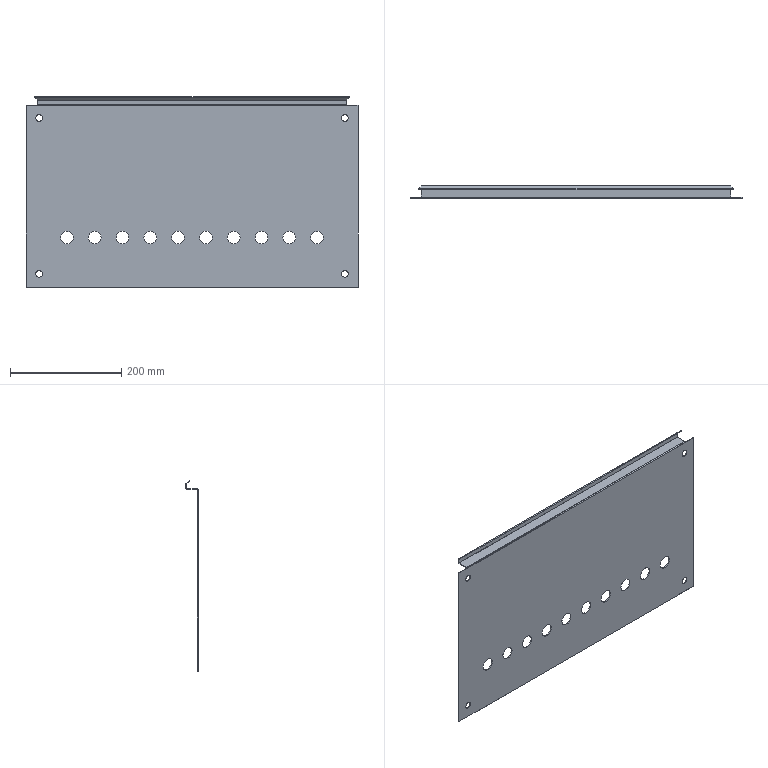Component | SolidWorks | BottomPlate-1 | 1 solid | 64 faces | volume 316921 mm3 | cylinder 34 | plane 28 | spline 2 | commonest cylinder face diameters 23 x20 12 x8 3.2 x3 0.2 x3